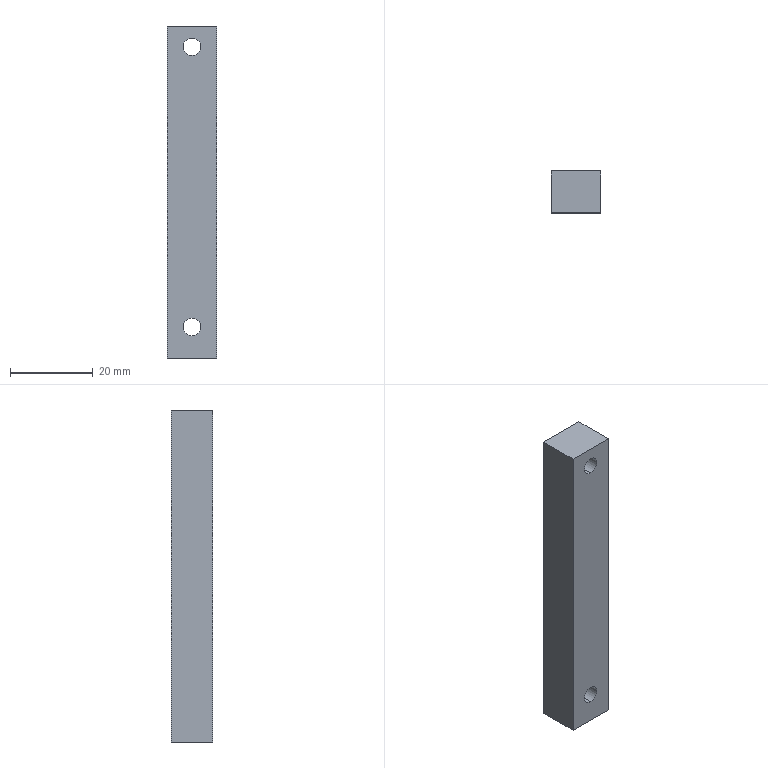Component | SolidWorks | RightLocatingPlate-1 | 1 solid | 10 faces | box 12 x 10 x 80 mm | volume 9323 mm3 | plane 6 | cylinder 4 | commonest cylinder face diameters 4.2 x4
build123d program:
from build123d import *

# Parameters (mm, degrees)
SKETCH1_W             = 80
SKETCH1_H             = 12
BOSS_EXTRUDE1_DEPTH   = 10
M5_TAPPED_HOLE1_D     = 4.2
M5_TAPPED_HOLE1_DEPTH = 14
M5_TAPPED_HOLE1_TIP   = 1.262
M5_TAPPED_HOLE2_D     = 4.2


with BuildPart() as part:
    # Sketch1 → Boss-Extrude1 (new body)
    with BuildSketch(Plane.XY):
        with Locations((40, 6)):
            Rectangle(SKETCH1_W, SKETCH1_H)
    extrude(amount=BOSS_EXTRUDE1_DEPTH)

    # M5 Tapped Hole1
    with Locations(Plane(origin=(72.5, 6, 10), x_dir=(1, 0, 0), z_dir=(0, 0, 1))):
        with Locations((0, 0)):
            Hole(M5_TAPPED_HOLE1_D / 2, depth=M5_TAPPED_HOLE1_DEPTH)
            with Locations((0, 0, -(M5_TAPPED_HOLE1_DEPTH + M5_TAPPED_HOLE1_TIP / 2))):  # 118° drill point
                Cone(0, M5_TAPPED_HOLE1_D / 2, M5_TAPPED_HOLE1_TIP, mode=Mode.SUBTRACT)

    # M5 Tapped Hole2 (through all)
    with Locations(Plane(origin=(5, 6, 0), x_dir=(-1, 0, 0), z_dir=(0, 0, -1))):
        with Locations((0, 0)):
            Hole(M5_TAPPED_HOLE2_D / 2)


solid = part.part

# Placed as in the assembly
solid = solid.moved(Location((134, -200.728, 136), (90, 0, -90)))
STEP:
#1=COLOUR_RGB('',0.7922,0.8196,0.9333);
#2=FILL_AREA_STYLE_COLOUR('',#1);
#3=FILL_AREA_STYLE('',(#2));
#4=SURFACE_STYLE_FILL_AREA(#3);
#5=SURFACE_SIDE_STYLE('',(#4));
#6=SURFACE_STYLE_USAGE(.BOTH.,#5);
#7=PRESENTATION_STYLE_ASSIGNMENT((#6));
#8=CARTESIAN_POINT('',(5.512,-7.903,5.075));
#9=VERTEX_POINT('',#8);
#10=CARTESIAN_POINT('',(5.512,-7.903,5.24));
#11=VERTEX_POINT('',#10);
#12=CARTESIAN_POINT('',(5.512,-7.903,5.157));
#13=DIRECTION('',(-0.,-1.,-0.));
#14=DIRECTION('',(0.,0.,1.));
#15=AXIS2_PLACEMENT_3D('',#12,#13,#14);
#16=CIRCLE('',#15,0.08268);
#17=EDGE_CURVE('',#9,#11,#16,.T.);
#18=ORIENTED_EDGE('',*,*,#17,.F.);
#19=CARTESIAN_POINT('',(5.512,-8.296,5.075));
#20=VERTEX_POINT('',#19);
#21=CARTESIAN_POINT('',(5.512,-8.296,5.075));
#22=DIRECTION('',(-0.,-1.,-0.));
#23=VECTOR('',#22,39.37);
#24=LINE('',#21,#23);
#25=EDGE_CURVE('',#9,#20,#24,.T.);
#26=ORIENTED_EDGE('',*,*,#25,.T.);
#27=CARTESIAN_POINT('',(5.512,-8.296,5.24));
#28=VERTEX_POINT('',#27);
#29=CARTESIAN_POINT('',(5.512,-8.296,5.157));
#30=DIRECTION('',(-0.,-1.,-0.));
#31=DIRECTION('',(0.,0.,1.));
#32=AXIS2_PLACEMENT_3D('',#29,#30,#31);
#33=CIRCLE('',#32,0.08268);
#34=EDGE_CURVE('',#20,#28,#33,.T.);
#35=ORIENTED_EDGE('',*,*,#34,.T.);
#36=CARTESIAN_POINT('',(5.512,-8.296,5.24));
#37=DIRECTION('',(-0.,-1.,-0.));
#38=VECTOR('',#37,39.37);
#39=LINE('',#36,#38);
#40=EDGE_CURVE('',#11,#28,#39,.T.);
#41=ORIENTED_EDGE('',*,*,#40,.F.);
#42=EDGE_LOOP('',(#18,#26,#35,#41));
#43=FACE_OUTER_BOUND('',#42,.T.);
#44=CARTESIAN_POINT('',(5.512,-8.296,5.157));
#45=DIRECTION('',(-0.,-1.,-0.));
#46=DIRECTION('',(0.,0.,1.));
#47=AXIS2_PLACEMENT_3D('',#44,#45,#46);
#48=CYLINDRICAL_SURFACE('',#47,0.08268);
#49=ADVANCED_FACE('',(#43),#48,.F.);
#50=CARTESIAN_POINT('',(5.512,-8.296,2.417));
#51=VERTEX_POINT('',#50);
#52=CARTESIAN_POINT('',(5.512,-8.296,2.583));
#53=VERTEX_POINT('',#52);
#54=CARTESIAN_POINT('',(5.512,-8.296,2.5));
#55=DIRECTION('',(-0.,-1.,-0.));
#56=DIRECTION('',(0.,0.,1.));
#57=AXIS2_PLACEMENT_3D('',#54,#55,#56);
#58=CIRCLE('',#57,0.08268);
#59=EDGE_CURVE('',#51,#53,#58,.T.);
#60=ORIENTED_EDGE('',*,*,#59,.T.);
#61=CARTESIAN_POINT('',(5.512,-7.903,2.583));
#62=VERTEX_POINT('',#61);
#63=CARTESIAN_POINT('',(5.512,-7.903,2.583));
#64=DIRECTION('',(0.,1.,0.));
#65=VECTOR('',#64,39.37);
#66=LINE('',#63,#65);
#67=EDGE_CURVE('',#53,#62,#66,.T.);
#68=ORIENTED_EDGE('',*,*,#67,.T.);
#69=CARTESIAN_POINT('',(5.512,-7.903,2.417));
#70=VERTEX_POINT('',#69);
#71=CARTESIAN_POINT('',(5.512,-7.903,2.5));
#72=DIRECTION('',(0.,1.,0.));
#73=DIRECTION('',(0.,0.,-1.));
#74=AXIS2_PLACEMENT_3D('',#71,#72,#73);
#75=CIRCLE('',#74,0.08268);
#76=EDGE_CURVE('',#62,#70,#75,.T.);
#77=ORIENTED_EDGE('',*,*,#76,.T.);
#78=CARTESIAN_POINT('',(5.512,-7.903,2.417));
#79=DIRECTION('',(0.,1.,0.));
#80=VECTOR('',#79,39.37);
#81=LINE('',#78,#80);
#82=EDGE_CURVE('',#51,#70,#81,.T.);
#83=ORIENTED_EDGE('',*,*,#82,.F.);
#84=EDGE_LOOP('',(#60,#68,#77,#83));
#85=FACE_OUTER_BOUND('',#84,.T.);
#86=CARTESIAN_POINT('',(5.512,-7.903,2.5));
#87=DIRECTION('',(0.,1.,0.));
#88=DIRECTION('',(0.,0.,-1.));
#89=AXIS2_PLACEMENT_3D('',#86,#87,#88);
#90=CYLINDRICAL_SURFACE('',#89,0.08268);
#91=ADVANCED_FACE('',(#85),#90,.F.);
#92=CARTESIAN_POINT('',(5.276,-8.296,5.354));
#93=VERTEX_POINT('',#92);
#94=CARTESIAN_POINT('',(5.748,-8.296,5.354));
#95=VERTEX_POINT('',#94);
#96=CARTESIAN_POINT('',(5.748,-8.296,5.354));
#97=DIRECTION('',(1.,-0.,0.));
#98=VECTOR('',#97,39.37);
#99=LINE('',#96,#98);
#100=EDGE_CURVE('',#93,#95,#99,.T.);
#101=ORIENTED_EDGE('',*,*,#100,.T.);
#102=CARTESIAN_POINT('',(5.748,-7.903,5.354));
#103=VERTEX_POINT('',#102);
#104=CARTESIAN_POINT('',(5.748,-7.903,5.354));
#105=DIRECTION('',(-0.,-1.,-0.));
#106=VECTOR('',#105,39.37);
#107=LINE('',#104,#106);
#108=EDGE_CURVE('',#103,#95,#107,.T.);
#109=ORIENTED_EDGE('',*,*,#108,.F.);
#110=CARTESIAN_POINT('',(5.276,-7.903,5.354));
#111=VERTEX_POINT('',#110);
#112=CARTESIAN_POINT('',(5.748,-7.903,5.354));
#113=DIRECTION('',(1.,-0.,0.));
#114=VECTOR('',#113,39.37);
#115=LINE('',#112,#114);
#116=EDGE_CURVE('',#111,#103,#115,.T.);
#117=ORIENTED_EDGE('',*,*,#116,.F.);
#118=CARTESIAN_POINT('',(5.276,-7.903,5.354));
#119=DIRECTION('',(-0.,-1.,-0.));
#120=VECTOR('',#119,39.37);
#121=LINE('',#118,#120);
#122=EDGE_CURVE('',#111,#93,#121,.T.);
#123=ORIENTED_EDGE('',*,*,#122,.T.);
#124=EDGE_LOOP('',(#101,#109,#117,#123));
#125=FACE_OUTER_BOUND('',#124,.T.);
#126=CARTESIAN_POINT('',(5.748,-7.903,5.354));
#127=DIRECTION('',(0.,0.,-1.));
#128=DIRECTION('',(-0.,-1.,-0.));
#129=AXIS2_PLACEMENT_3D('',#126,#127,#128);
#130=PLANE('',#129);
#131=ADVANCED_FACE('',(#125),#130,.F.);
#132=CARTESIAN_POINT('',(5.748,-8.296,2.205));
#133=VERTEX_POINT('',#132);
#134=CARTESIAN_POINT('',(5.748,-8.296,5.354));
#135=DIRECTION('',(0.,0.,-1.));
#136=VECTOR('',#135,39.37);
#137=LINE('',#134,#136);
#138=EDGE_CURVE('',#95,#133,#137,.T.);
#139=ORIENTED_EDGE('',*,*,#138,.T.);
#140=CARTESIAN_POINT('',(5.748,-7.903,2.205));
#141=VERTEX_POINT('',#140);
#142=CARTESIAN_POINT('',(5.748,-7.903,2.205));
#143=DIRECTION('',(-0.,-1.,-0.));
#144=VECTOR('',#143,39.37);
#145=LINE('',#142,#144);
#146=EDGE_CURVE('',#141,#133,#145,.T.);
#147=ORIENTED_EDGE('',*,*,#146,.F.);
#148=CARTESIAN_POINT('',(5.748,-7.903,5.354));
#149=DIRECTION('',(0.,0.,-1.));
#150=VECTOR('',#149,39.37);
#151=LINE('',#148,#150);
#152=EDGE_CURVE('',#103,#141,#151,.T.);
#153=ORIENTED_EDGE('',*,*,#152,.F.);
#154=ORIENTED_EDGE('',*,*,#108,.T.);
#155=EDGE_LOOP('',(#139,#147,#153,#154));
#156=FACE_OUTER_BOUND('',#155,.T.);
#157=CARTESIAN_POINT('',(5.748,-7.903,5.354));
#158=DIRECTION('',(-1.,0.,-0.));
#159=DIRECTION('',(0.,1.,0.));
#160=AXIS2_PLACEMENT_3D('',#157,#158,#159);
#161=PLANE('',#160);
#162=ADVANCED_FACE('',(#156),#161,.F.);
#163=CARTESIAN_POINT('',(5.276,-8.296,2.205));
#164=VERTEX_POINT('',#163);
#165=CARTESIAN_POINT('',(5.748,-8.296,2.205));
#166=DIRECTION('',(-1.,0.,-0.));
#167=VECTOR('',#166,39.37);
#168=LINE('',#165,#167);
#169=EDGE_CURVE('',#133,#164,#168,.T.);
#170=ORIENTED_EDGE('',*,*,#169,.T.);
#171=CARTESIAN_POINT('',(5.276,-7.903,2.205));
#172=VERTEX_POINT('',#171);
#173=CARTESIAN_POINT('',(5.276,-7.903,2.205));
#174=DIRECTION('',(-0.,-1.,-0.));
#175=VECTOR('',#174,39.37);
#176=LINE('',#173,#175);
#177=EDGE_CURVE('',#172,#164,#176,.T.);
#178=ORIENTED_EDGE('',*,*,#177,.F.);
#179=CARTESIAN_POINT('',(5.748,-7.903,2.205));
#180=DIRECTION('',(-1.,0.,-0.));
#181=VECTOR('',#180,39.37);
#182=LINE('',#179,#181);
#183=EDGE_CURVE('',#141,#172,#182,.T.);
#184=ORIENTED_EDGE('',*,*,#183,.F.);
#185=ORIENTED_EDGE('',*,*,#146,.T.);
#186=EDGE_LOOP('',(#170,#178,#184,#185));
#187=FACE_OUTER_BOUND('',#186,.T.);
#188=CARTESIAN_POINT('',(5.748,-7.903,2.205));
#189=DIRECTION('',(-0.,-0.,1.));
#190=DIRECTION('',(0.,1.,0.));
#191=AXIS2_PLACEMENT_3D('',#188,#189,#190);
#192=PLANE('',#191);
#193=ADVANCED_FACE('',(#187),#192,.F.);
#194=CARTESIAN_POINT('',(5.276,-8.296,5.354));
#195=DIRECTION('',(-0.,-0.,1.));
#196=VECTOR('',#195,39.37);
#197=LINE('',#194,#196);
#198=EDGE_CURVE('',#164,#93,#197,.T.);
#199=ORIENTED_EDGE('',*,*,#198,.T.);
#200=ORIENTED_EDGE('',*,*,#122,.F.);
#201=CARTESIAN_POINT('',(5.276,-7.903,5.354));
#202=DIRECTION('',(-0.,-0.,1.));
#203=VECTOR('',#202,39.37);
#204=LINE('',#201,#203);
#205=EDGE_CURVE('',#172,#111,#204,.T.);
#206=ORIENTED_EDGE('',*,*,#205,.F.);
#207=ORIENTED_EDGE('',*,*,#177,.T.);
#208=EDGE_LOOP('',(#199,#200,#206,#207));
#209=FACE_OUTER_BOUND('',#208,.T.);
#210=CARTESIAN_POINT('',(5.276,-7.903,5.354));
#211=DIRECTION('',(1.,-0.,0.));
#212=DIRECTION('',(-0.,-1.,-0.));
#213=AXIS2_PLACEMENT_3D('',#210,#211,#212);
#214=PLANE('',#213);
#215=ADVANCED_FACE('',(#209),#214,.F.);
#216=CARTESIAN_POINT('',(5.512,-7.903,5.157));
#217=DIRECTION('',(-0.,-1.,-0.));
#218=DIRECTION('',(0.,0.,1.));
#219=AXIS2_PLACEMENT_3D('',#216,#217,#218);
#220=CIRCLE('',#219,0.08268);
#221=EDGE_CURVE('',#11,#9,#220,.T.);
#222=ORIENTED_EDGE('',*,*,#221,.T.);
#223=ORIENTED_EDGE('',*,*,#17,.T.);
#224=EDGE_LOOP('',(#222,#223));
#225=FACE_BOUND('',#224,.T.);
#226=CARTESIAN_POINT('',(5.512,-7.903,2.5));
#227=DIRECTION('',(0.,1.,0.));
#228=DIRECTION('',(0.,0.,-1.));
#229=AXIS2_PLACEMENT_3D('',#226,#227,#228);
#230=CIRCLE('',#229,0.08268);
#231=EDGE_CURVE('',#70,#62,#230,.T.);
#232=ORIENTED_EDGE('',*,*,#231,.F.);
#233=ORIENTED_EDGE('',*,*,#76,.F.);
#234=EDGE_LOOP('',(#232,#233));
#235=FACE_BOUND('',#234,.T.);
#236=ORIENTED_EDGE('',*,*,#116,.T.);
#237=ORIENTED_EDGE('',*,*,#152,.T.);
#238=ORIENTED_EDGE('',*,*,#183,.T.);
#239=ORIENTED_EDGE('',*,*,#205,.T.);
#240=EDGE_LOOP('',(#236,#237,#238,#239));
#241=FACE_OUTER_BOUND('',#240,.T.);
#242=CARTESIAN_POINT('',(5.748,-7.903,5.354));
#243=DIRECTION('',(-0.,-1.,-0.));
#244=DIRECTION('',(-0.,-0.,1.));
#245=AXIS2_PLACEMENT_3D('',#242,#243,#244);
#246=PLANE('',#245);
#247=ADVANCED_FACE('',(#225,#235,#241),#246,.F.);
#248=CARTESIAN_POINT('',(5.512,-8.296,5.157));
#249=DIRECTION('',(-0.,-1.,-0.));
#250=DIRECTION('',(0.,0.,1.));
#251=AXIS2_PLACEMENT_3D('',#248,#249,#250);
#252=CIRCLE('',#251,0.08268);
#253=EDGE_CURVE('',#28,#20,#252,.T.);
#254=ORIENTED_EDGE('',*,*,#253,.F.);
#255=ORIENTED_EDGE('',*,*,#34,.F.);
#256=EDGE_LOOP('',(#254,#255));
#257=FACE_BOUND('',#256,.T.);
#258=ORIENTED_EDGE('',*,*,#59,.F.);
#259=CARTESIAN_POINT('',(5.512,-8.296,2.5));
#260=DIRECTION('',(-0.,-1.,-0.));
#261=DIRECTION('',(0.,0.,1.));
#262=AXIS2_PLACEMENT_3D('',#259,#260,#261);
#263=CIRCLE('',#262,0.08268);
#264=EDGE_CURVE('',#53,#51,#263,.T.);
#265=ORIENTED_EDGE('',*,*,#264,.F.);
#266=EDGE_LOOP('',(#258,#265));
#267=FACE_BOUND('',#266,.T.);
#268=ORIENTED_EDGE('',*,*,#100,.F.);
#269=ORIENTED_EDGE('',*,*,#198,.F.);
#270=ORIENTED_EDGE('',*,*,#169,.F.);
#271=ORIENTED_EDGE('',*,*,#138,.F.);
#272=EDGE_LOOP('',(#268,#269,#270,#271));
#273=FACE_OUTER_BOUND('',#272,.T.);
#274=CARTESIAN_POINT('',(5.748,-8.296,5.354));
#275=DIRECTION('',(-0.,-1.,-0.));
#276=DIRECTION('',(-0.,-0.,1.));
#277=AXIS2_PLACEMENT_3D('',#274,#275,#276);
#278=PLANE('',#277);
#279=ADVANCED_FACE('',(#257,#267,#273),#278,.T.);
#280=ORIENTED_EDGE('',*,*,#67,.F.);
#281=ORIENTED_EDGE('',*,*,#264,.T.);
#282=ORIENTED_EDGE('',*,*,#82,.T.);
#283=ORIENTED_EDGE('',*,*,#231,.T.);
#284=EDGE_LOOP('',(#280,#281,#282,#283));
#285=FACE_OUTER_BOUND('',#284,.T.);
#286=CARTESIAN_POINT('',(5.512,-7.903,2.5));
#287=DIRECTION('',(0.,1.,0.));
#288=DIRECTION('',(0.,0.,-1.));
#289=AXIS2_PLACEMENT_3D('',#286,#287,#288);
#290=CYLINDRICAL_SURFACE('',#289,0.08268);
#291=ADVANCED_FACE('',(#285),#290,.F.);
#292=ORIENTED_EDGE('',*,*,#25,.F.);
#293=ORIENTED_EDGE('',*,*,#221,.F.);
#294=ORIENTED_EDGE('',*,*,#40,.T.);
#295=ORIENTED_EDGE('',*,*,#253,.T.);
#296=EDGE_LOOP('',(#292,#293,#294,#295));
#297=FACE_OUTER_BOUND('',#296,.T.);
#298=CARTESIAN_POINT('',(5.512,-8.296,5.157));
#299=DIRECTION('',(-0.,-1.,-0.));
#300=DIRECTION('',(0.,0.,1.));
#301=AXIS2_PLACEMENT_3D('',#298,#299,#300);
#302=CYLINDRICAL_SURFACE('',#301,0.08268);
#303=ADVANCED_FACE('',(#297),#302,.F.);
#304=CLOSED_SHELL('',(#49,#91,#131,#162,#193,#215,#247,#279,#291,#303));
#305=MANIFOLD_SOLID_BREP('',#304);
#306=STYLED_ITEM('',(#7),#305);
#307=PRESENTATION_LAYER_ASSIGNMENT('','',(#306));
#308=(LENGTH_UNIT()NAMED_UNIT(*)SI_UNIT($,.METRE.));
#309=LENGTH_MEASURE_WITH_UNIT(LENGTH_MEASURE(0.0254),#308);
#310=DIMENSIONAL_EXPONENTS(1.,0.,0.,0.,0.,0.,0.);
#311=(CONVERSION_BASED_UNIT('',#309)LENGTH_UNIT()NAMED_UNIT(#310));
#312=UNCERTAINTY_MEASURE_WITH_UNIT(LENGTH_MEASURE(0.00001),#311,'','');
#313=(NAMED_UNIT(*)PLANE_ANGLE_UNIT()SI_UNIT($,.RADIAN.));
#314=(NAMED_UNIT(*)SI_UNIT($,.STERADIAN.)SOLID_ANGLE_UNIT());
#315=(GEOMETRIC_REPRESENTATION_CONTEXT(3)GLOBAL_UNCERTAINTY_ASSIGNED_CONTEXT((#312))GLOBAL_UNIT_ASSIGNED_CONTEXT((#311,#313,#314))REPRESENTATION_CONTEXT('',''));
#316=MECHANICAL_DESIGN_GEOMETRIC_PRESENTATION_REPRESENTATION('',(#306),#315);
#317=CARTESIAN_POINT('',(0.,0.,0.));
#318=DIRECTION('',(0.,0.,1.));
#319=DIRECTION('',(1.,0.,0.));
#320=AXIS2_PLACEMENT_3D('',#317,#318,#319);
#321=(LENGTH_UNIT()NAMED_UNIT(*)SI_UNIT($,.METRE.));
#322=LENGTH_MEASURE_WITH_UNIT(LENGTH_MEASURE(0.0254),#321);
#323=DIMENSIONAL_EXPONENTS(1.,0.,0.,0.,0.,0.,0.);
#324=(CONVERSION_BASED_UNIT('',#322)LENGTH_UNIT()NAMED_UNIT(#323));
#325=UNCERTAINTY_MEASURE_WITH_UNIT(LENGTH_MEASURE(0.00001),#324,'','');
#326=(NAMED_UNIT(*)PLANE_ANGLE_UNIT()SI_UNIT($,.RADIAN.));
#327=(NAMED_UNIT(*)SI_UNIT($,.STERADIAN.)SOLID_ANGLE_UNIT());
#328=(GEOMETRIC_REPRESENTATION_CONTEXT(3)GLOBAL_UNCERTAINTY_ASSIGNED_CONTEXT((#325))GLOBAL_UNIT_ASSIGNED_CONTEXT((#324,#326,#327))REPRESENTATION_CONTEXT('',''));
#329=ADVANCED_BREP_SHAPE_REPRESENTATION('',(#305,#320),#328);